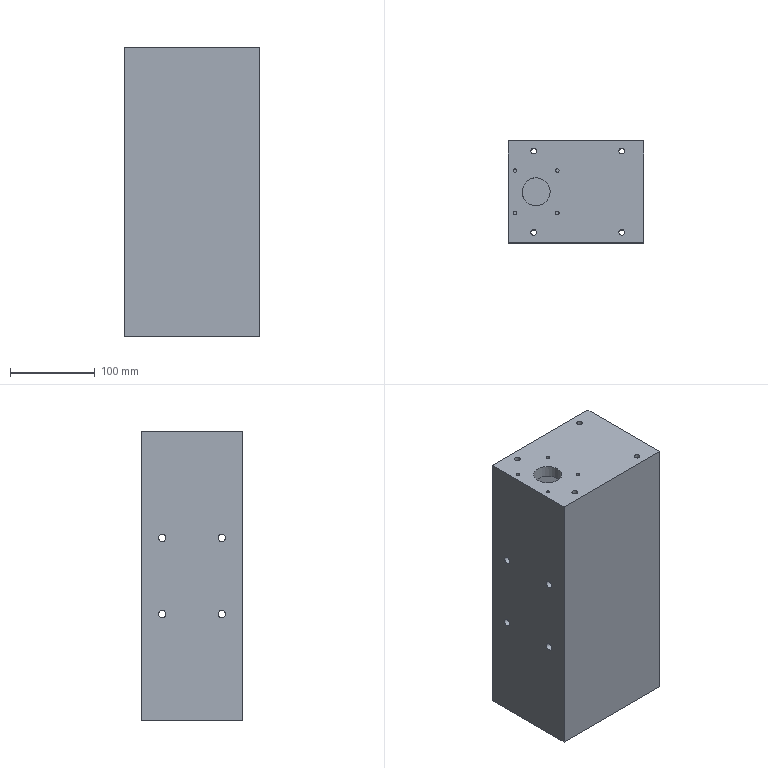Component | NX | Z_AXIS_HOUSING | 1 solid | 39 faces | volume 1612723 mm3 | cylinder 22 | plane 17 | commonest cylinder face diameters 6.8 x8 5 x4 4.2 x4 8.5 x4 50 x1 33 x1